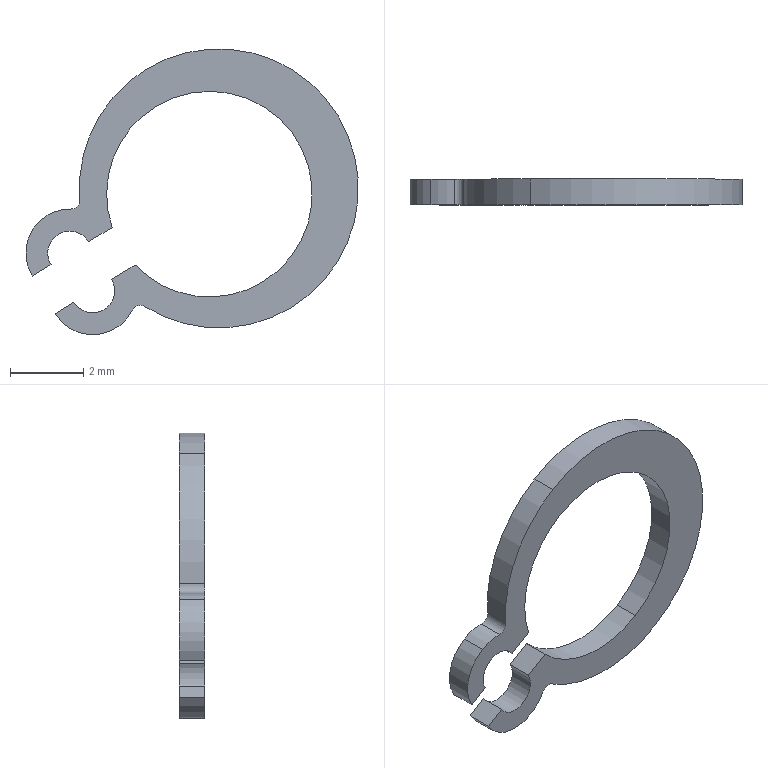Component | SolidWorks | JL001-03-06-4_GB_T894-2017[AxisElasticRetainingRingTypeA(d0_9)6]-1 | 1 solid | 21 faces | box 9.06 x 0.7 x 7.79 mm | volume 16 mm3 | cylinder 15 | plane 6 | commonest cylinder face diameters 7.6 x3 0.48 x3 5.6 x3 1.2 x3 2.4 x3
build123d program:
from build123d import *

# Parameters (mm, degrees)
EXTRUDE1_DEPTH = 0.7


with BuildPart() as part:
    # Dimension Sketch → Extrude1 (new body)
    with BuildSketch(Plane.XY):
        with BuildLine():
            Line((-0.6, -2.735), (-0.6, -3.485))
            ThreePointArc((-0.6, -3.485), (-1.2, -4.085), (-0.6, -4.685))
            Line((-0.6, -4.685), (-0.6, -5.285))
            ThreePointArc((-0.6, -5.285), (-1.652, -4.662), (-1.611, -3.439))
            ThreePointArc((-1.611, -3.439), (-1.582, -3.246), (-1.706, -3.096))
            ThreePointArc((-1.706, -3.096), (0, 4.1), (1.706, -3.096))
            ThreePointArc((1.706, -3.096), (1.582, -3.246), (1.611, -3.439))
            ThreePointArc((1.611, -3.439), (1.652, -4.662), (0.6, -5.285))
            Line((0.6, -5.285), (0.6, -4.685))
            ThreePointArc((0.6, -4.685), (1.2, -4.085), (0.6, -3.485))
            Line((0.6, -3.485), (0.6, -2.735))
            ThreePointArc((0.6, -2.735), (0, 2.8), (-0.6, -2.735))
        make_face()
    extrude(amount=EXTRUDE1_DEPTH)


solid = part.part

# Placed as in the assembly
solid = solid.moved(Location((-15, 48.5, 112.5), (-90, 0, -121.277)))